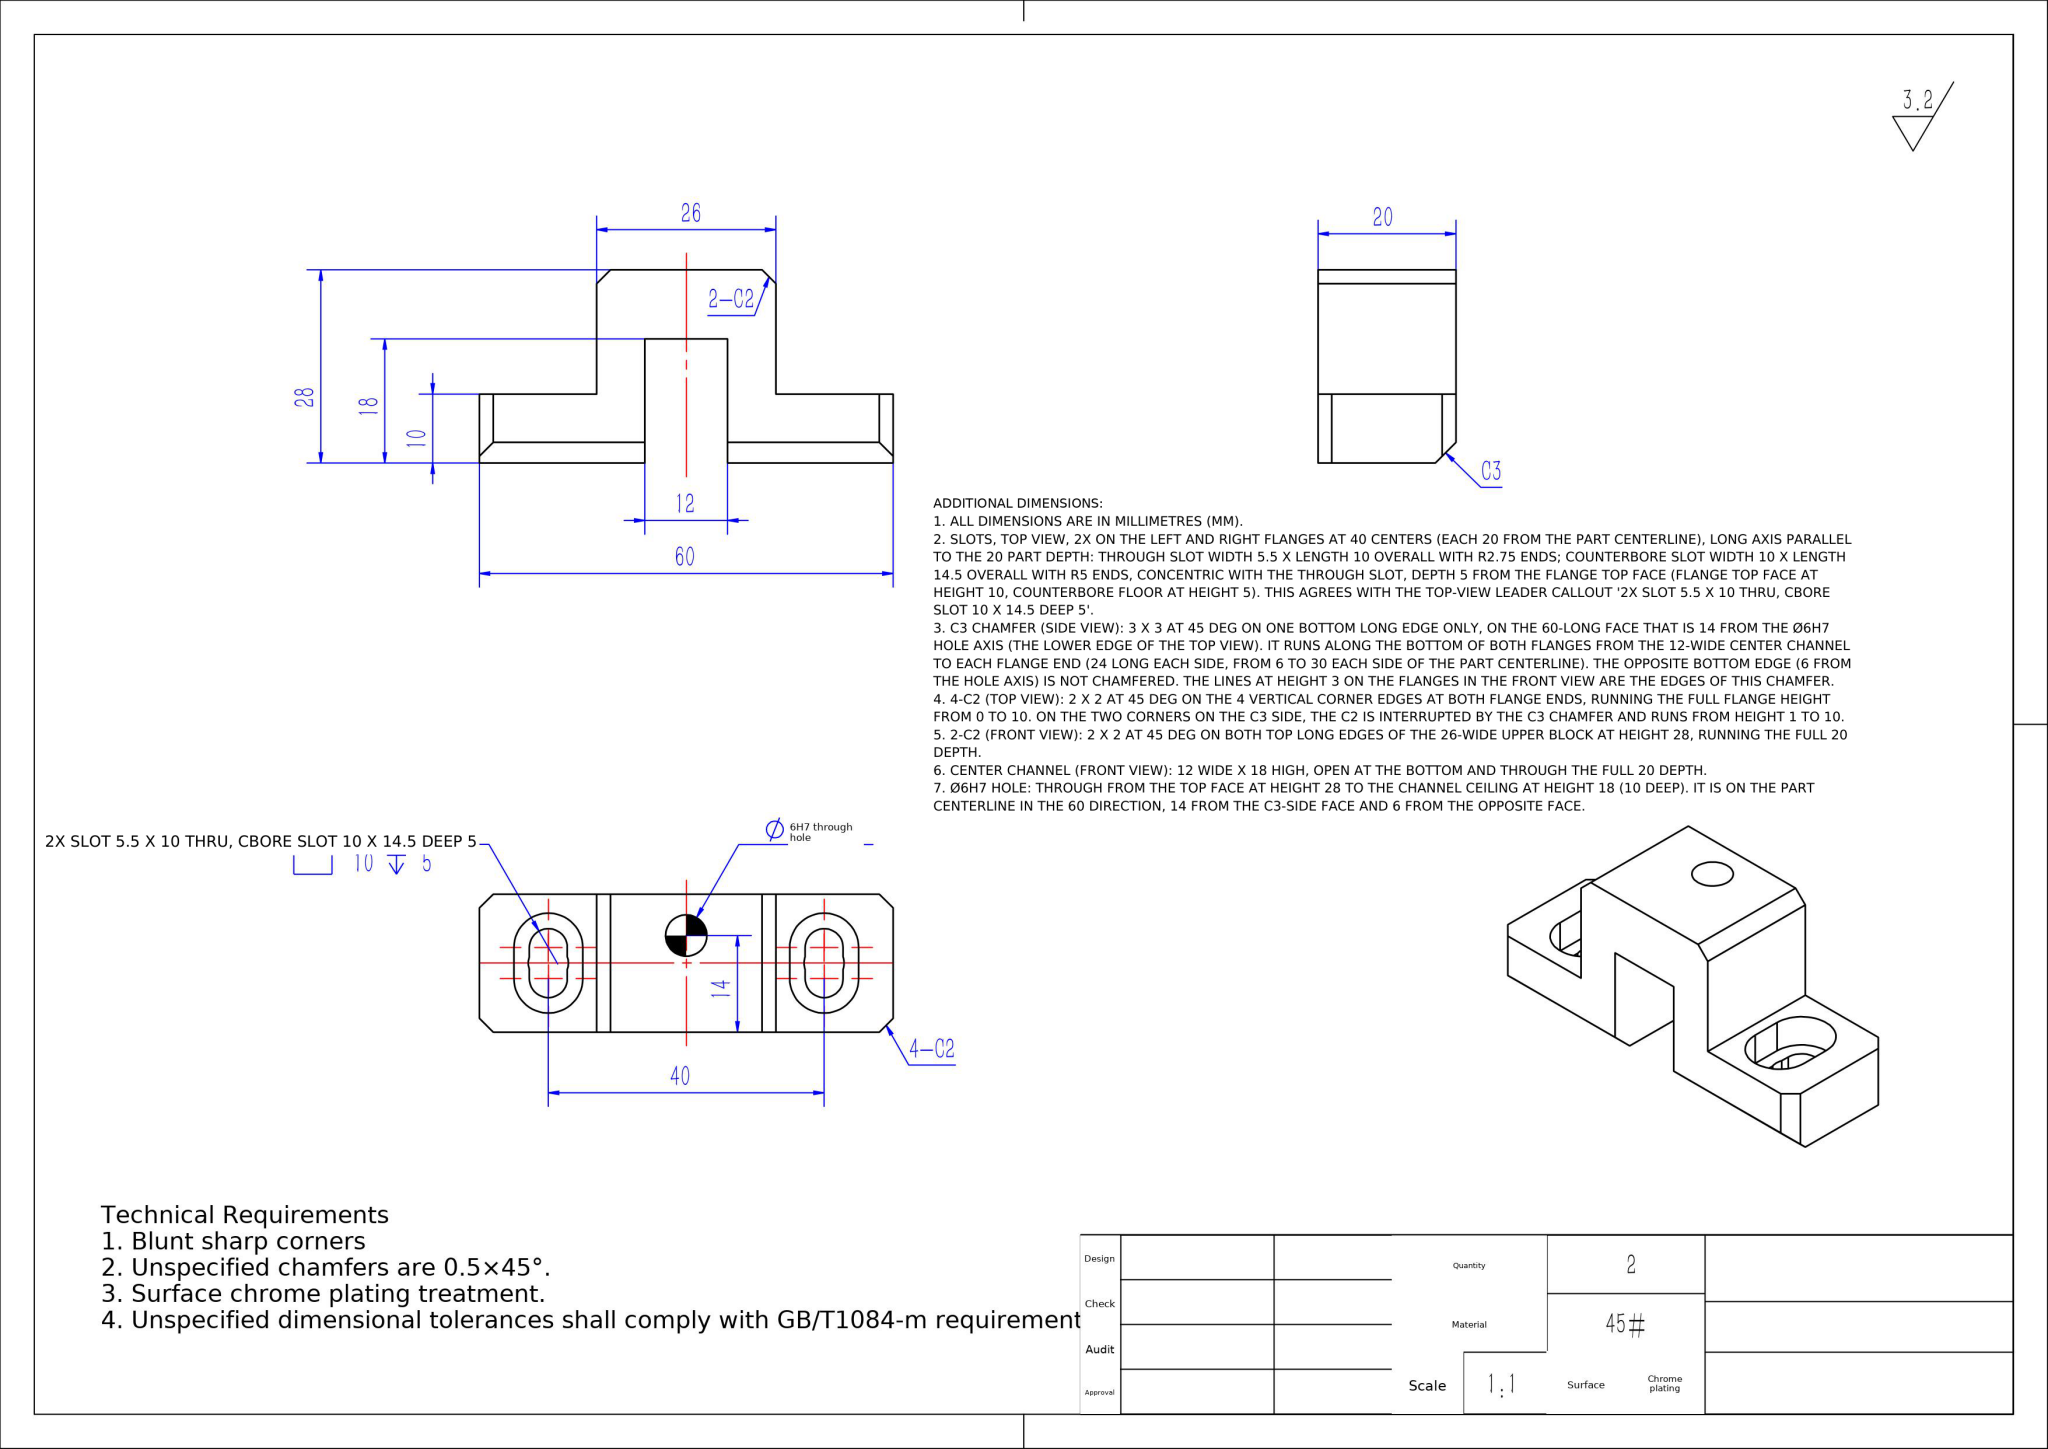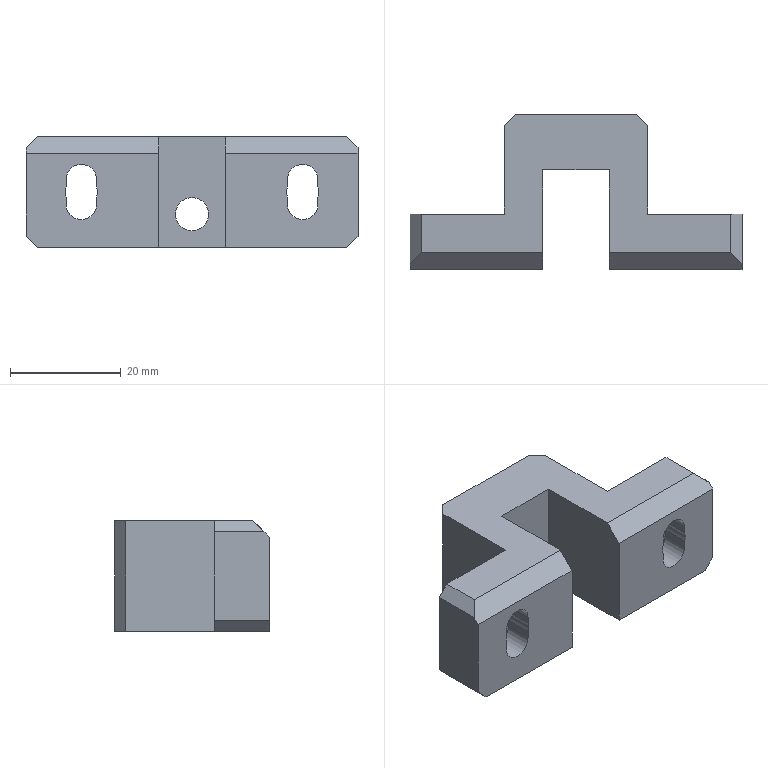Part | NX | mm | 1 solid | 54 faces | box 60 x 28 x 20 mm | volume 14666 mm3 | plane 36 | cylinder 18 | commonest cylinder face diameters 10 x6 5.5 x6 5.8 x4 6 x2